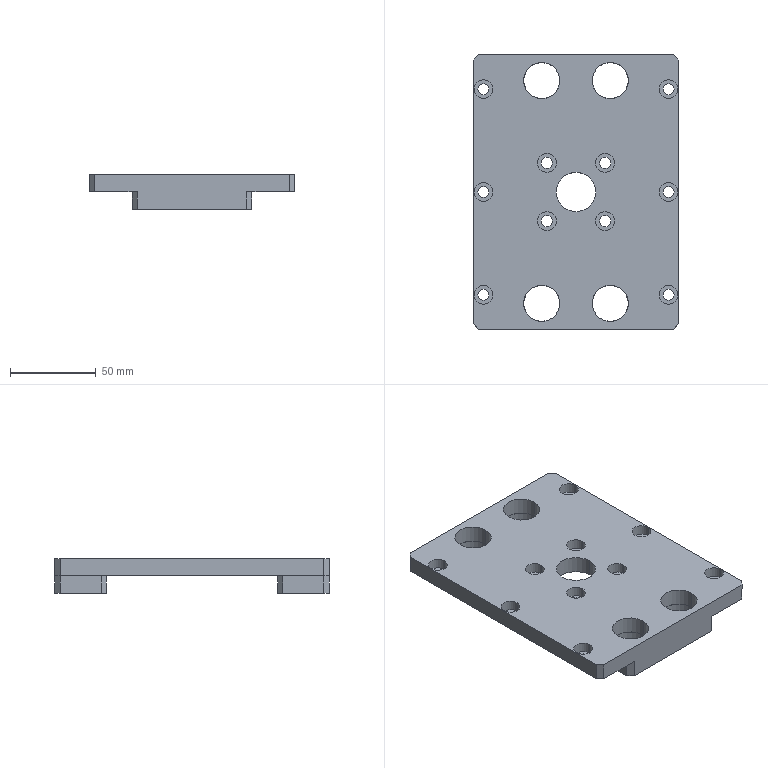Component | SolidWorks | A-C13SupportCylinderBasePlate-1 | 1 solid | 98 faces | box 120 x 160 x 20.3 mm | volume 195143 mm3 | cylinder 58 | plane 40 | commonest cylinder face diameters 11 x20 6.4 x12 21 x8 6.6 x8 21.2 x8 23 x2
build123d program:
from build123d import *

# Parameters (mm, degrees)
SKETCH1_W                                       = 120
SKETCH1_H                                       = 160
SKETCH1_R                                       = 10.6
EXTRUDE1_DEPTH                                  = 10
M6_HEX_SOCKET_HEAD_CAP_SCREW_CBORE1_D           = 6.6
M6_HEX_SOCKET_HEAD_CAP_SCREW_CBORE1_CBORE_D     = 11
M6_HEX_SOCKET_HEAD_CAP_SCREW_CBORE1_CBORE_DEPTH = 6
SKETCH11_R                                      = 11.5
EXTRUDE2_DEPTH                                  = 101.499
SKETCH12_W                                      = 70
SKETCH12_H                                      = 30
SKETCH12_R                                      = 10.5
BOSS_EXTRUDE1_DEPTH                             = 10.3
CHAMFER1_SIZE                                   = 3
M6_HEX_SOCKET_HEAD_CAP_SCREW_CBORE2_D           = 6.4
M6_HEX_SOCKET_HEAD_CAP_SCREW_CBORE2_CBORE_D     = 11
M6_HEX_SOCKET_HEAD_CAP_SCREW_CBORE2_CBORE_DEPTH = 6


with BuildPart() as part:
    # Sketch1 → Extrude1 (new body)
    with BuildSketch(Plane.XY):
        Rectangle(SKETCH1_W, SKETCH1_H)
        with Locations((20, 65)):
            Circle(SKETCH1_R, mode=Mode.SUBTRACT)
        with Locations(Location((-20, 65, 0), (0, 0, 180))):
            Circle(SKETCH1_R, mode=Mode.SUBTRACT)
        with Locations((-20, -65)):
            Circle(SKETCH1_R, mode=Mode.SUBTRACT)
        with Locations(Location((20, -65, 0), (0, 0, 180))):
            Circle(SKETCH1_R, mode=Mode.SUBTRACT)
    extrude(amount=EXTRUDE1_DEPTH)

    # M6 Hex Socket Head Cap Screw CBORE1 (through all)
    with Locations(Plane.XY.offset(10)):
        with Locations((17, 17), (-17, 17), (-17, -17), (17, -17)):
            CounterBoreHole(M6_HEX_SOCKET_HEAD_CAP_SCREW_CBORE1_D / 2, M6_HEX_SOCKET_HEAD_CAP_SCREW_CBORE1_CBORE_D / 2, M6_HEX_SOCKET_HEAD_CAP_SCREW_CBORE1_CBORE_DEPTH)

    # Sketch11 → Extrude2 (cut, through all)
    with BuildSketch(Plane.XY.offset(10)):
        Circle(SKETCH11_R)
    extrude(amount=-EXTRUDE2_DEPTH, mode=Mode.SUBTRACT)

    # Sketch12 → Boss-Extrude1 (add)
    # profile 1 of 2: a face of its own
    with BuildSketch(Plane(origin=(0, 0, 0), x_dir=(-1, 0, 0), z_dir=(0, 0, -1))):
        with Locations((0, 65)):
            Rectangle(SKETCH12_W, SKETCH12_H)
        with Locations(Location((-20, 65, 0), (0, 0, 180))):
            Circle(SKETCH12_R, mode=Mode.SUBTRACT)
        with Locations(Location((20, 65, 0), (0, 0, 180))):
            Circle(SKETCH12_R, mode=Mode.SUBTRACT)
    # profile 2 of 2: a face of its own
    with BuildSketch(Plane(origin=(0, 0, 0), x_dir=(-1, 0, 0), z_dir=(0, 0, -1))):
        with Locations((0, -65)):
            Rectangle(SKETCH12_W, SKETCH12_H)
        with Locations(Location((-20, -65, 0), (0, 0, 180))):
            Circle(SKETCH12_R, mode=Mode.SUBTRACT)
        with Locations(Location((20, -65, 0), (0, 0, 180))):
            Circle(SKETCH12_R, mode=Mode.SUBTRACT)
    extrude(amount=BOSS_EXTRUDE1_DEPTH)

    # Chamfer1
    chamfer1_edges = [part.edges().sort_by_distance(p)[0] for p in [
        (35, 80, -5.15),
        (35, 50, -5.15),
        (-35, 50, -5.15),
        (-35, 80, -5.15),
        (-60, 80, 5),
        (-60, -80, 5),
        (-35, -80, -5.15),
        (-35, -50, -5.15),
        (35, -50, -5.15),
        (35, -80, -5.15),
        (60, -80, 5),
        (60, 80, 5),
    ]]
    chamfer(chamfer1_edges, length=CHAMFER1_SIZE)

    # M6 Hex Socket Head Cap Screw CBORE2 (through all)
    with Locations(Plane.XY.offset(10)):
        with Locations((-54, -60), (-54, 0), (-54, 60), (54, -60), (54, 0), (54, 60)):
            CounterBoreHole(M6_HEX_SOCKET_HEAD_CAP_SCREW_CBORE2_D / 2, M6_HEX_SOCKET_HEAD_CAP_SCREW_CBORE2_CBORE_D / 2, M6_HEX_SOCKET_HEAD_CAP_SCREW_CBORE2_CBORE_DEPTH)


solid = part.part

# Placed as in the assembly
solid = solid.moved(Location((-33.181, 22.568, 0), (0, 0, 0)))